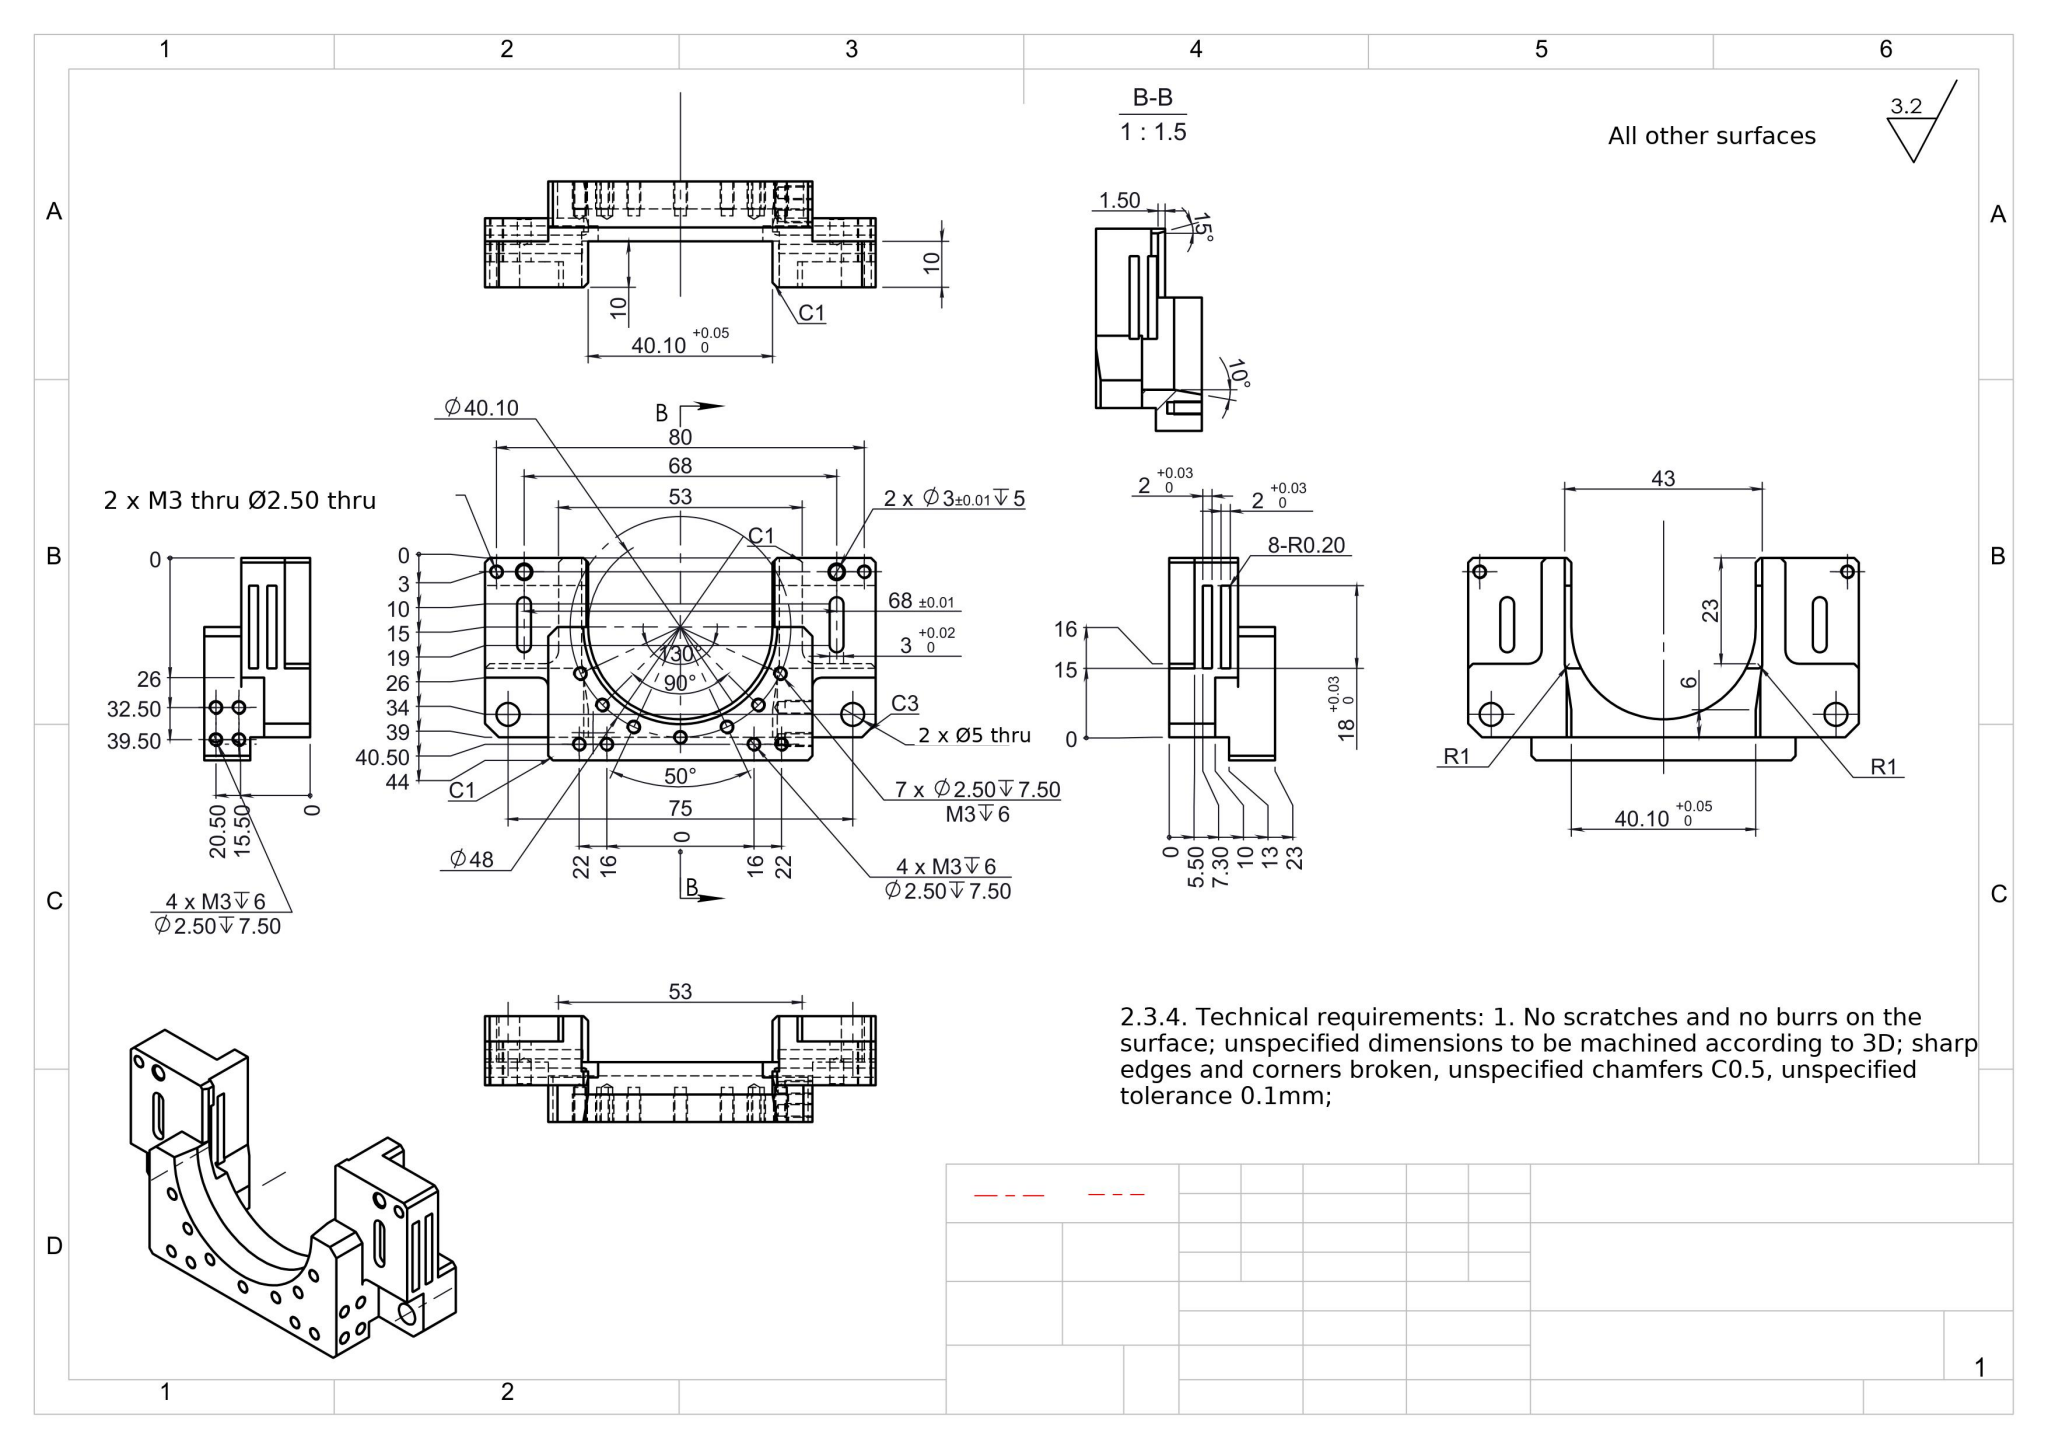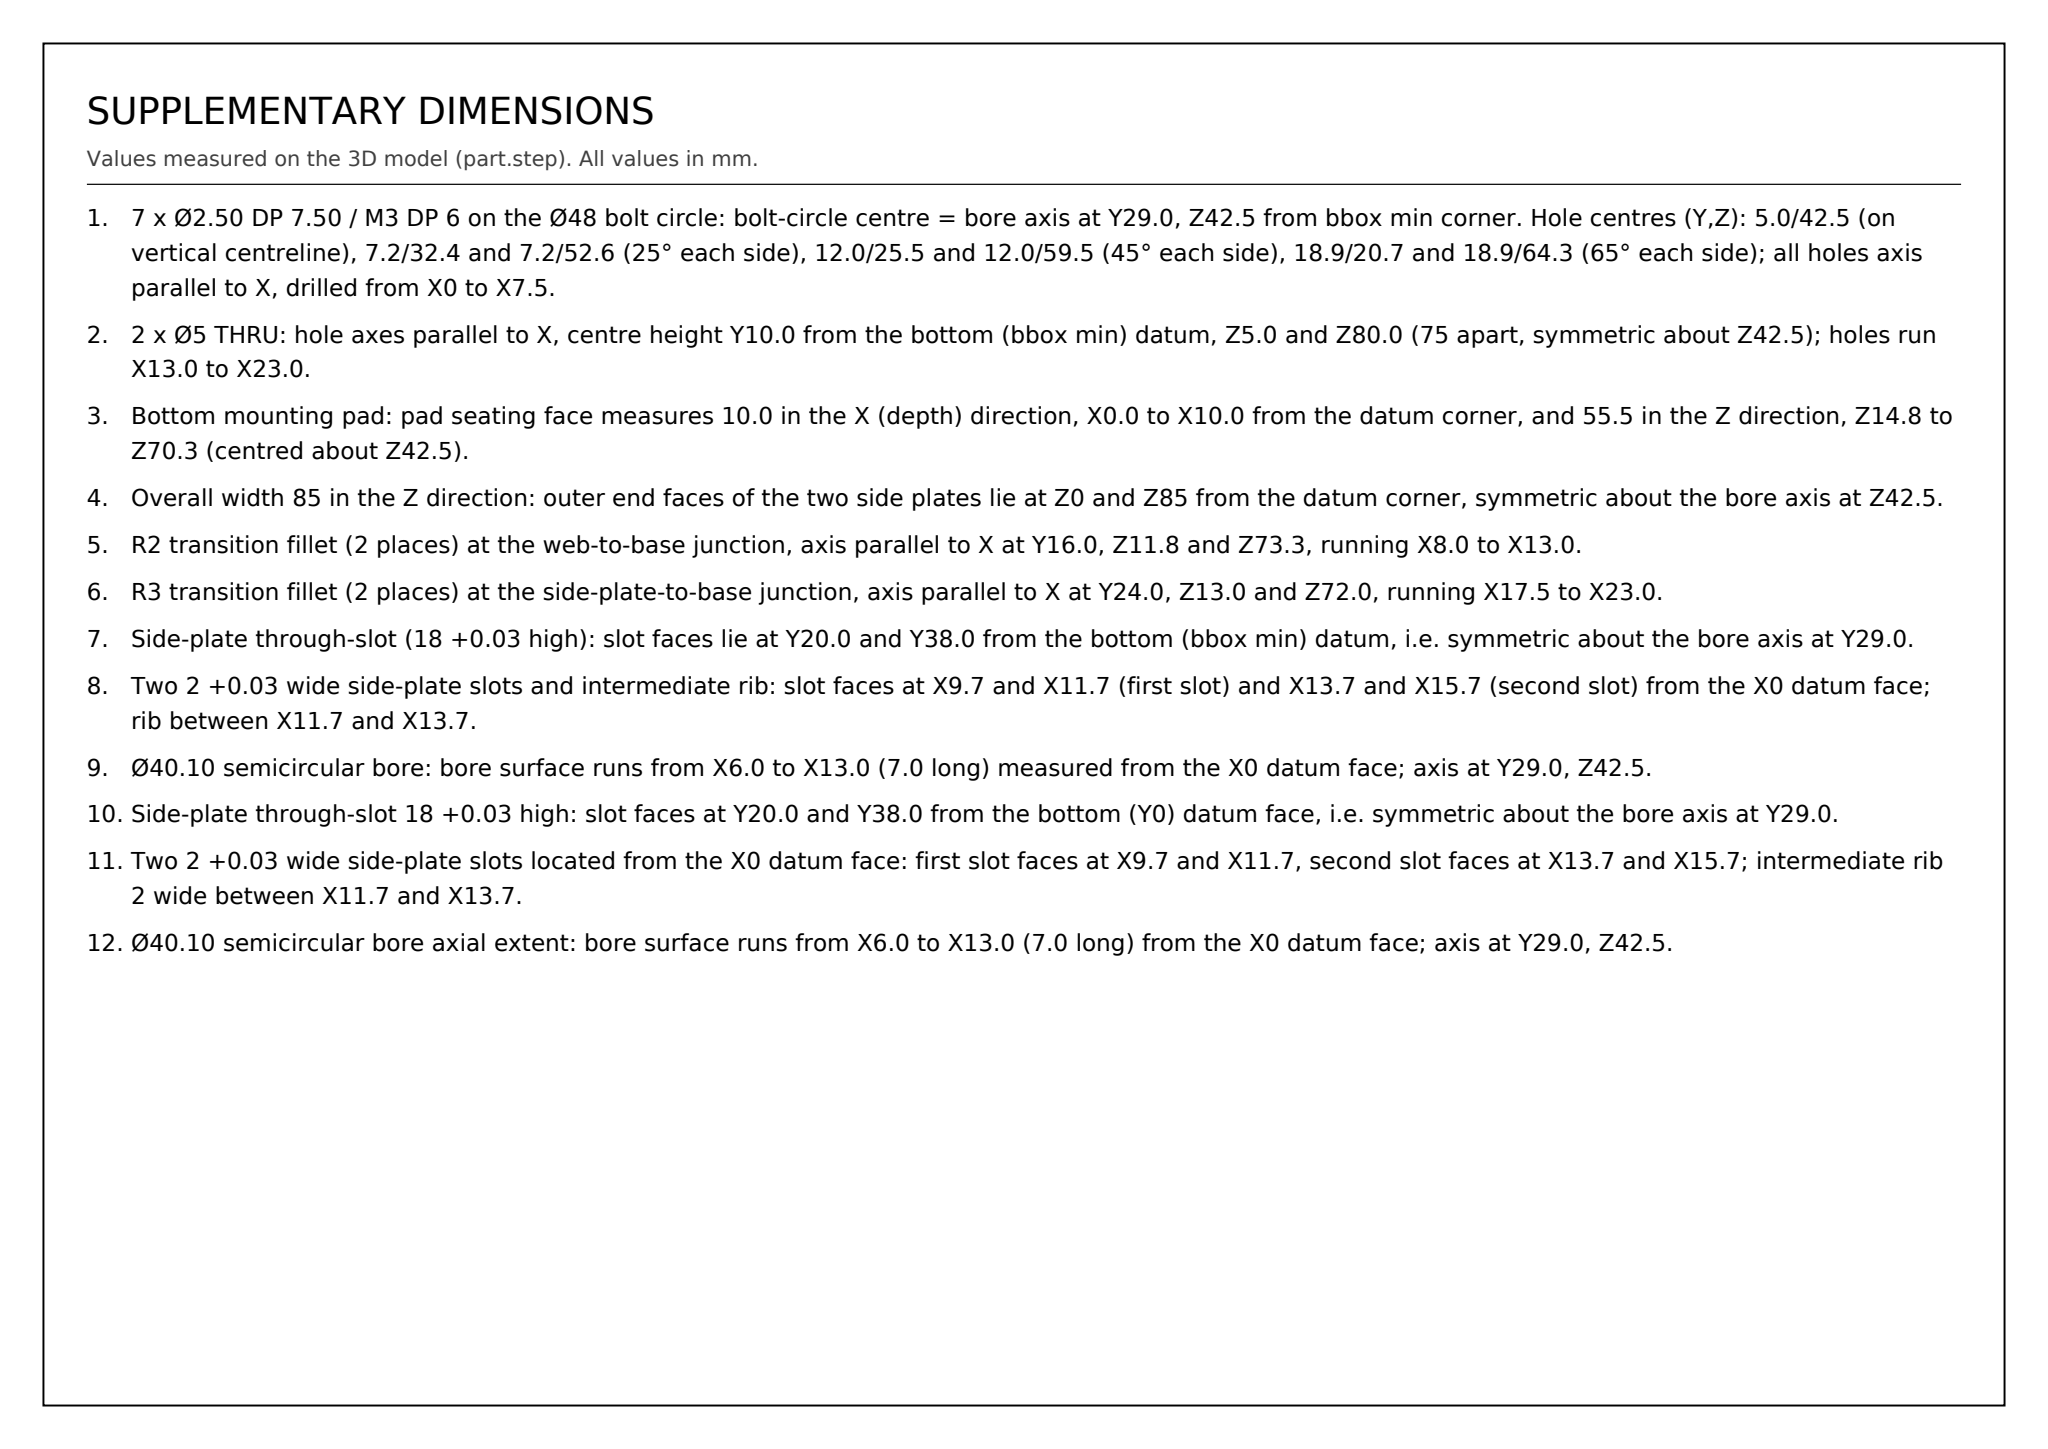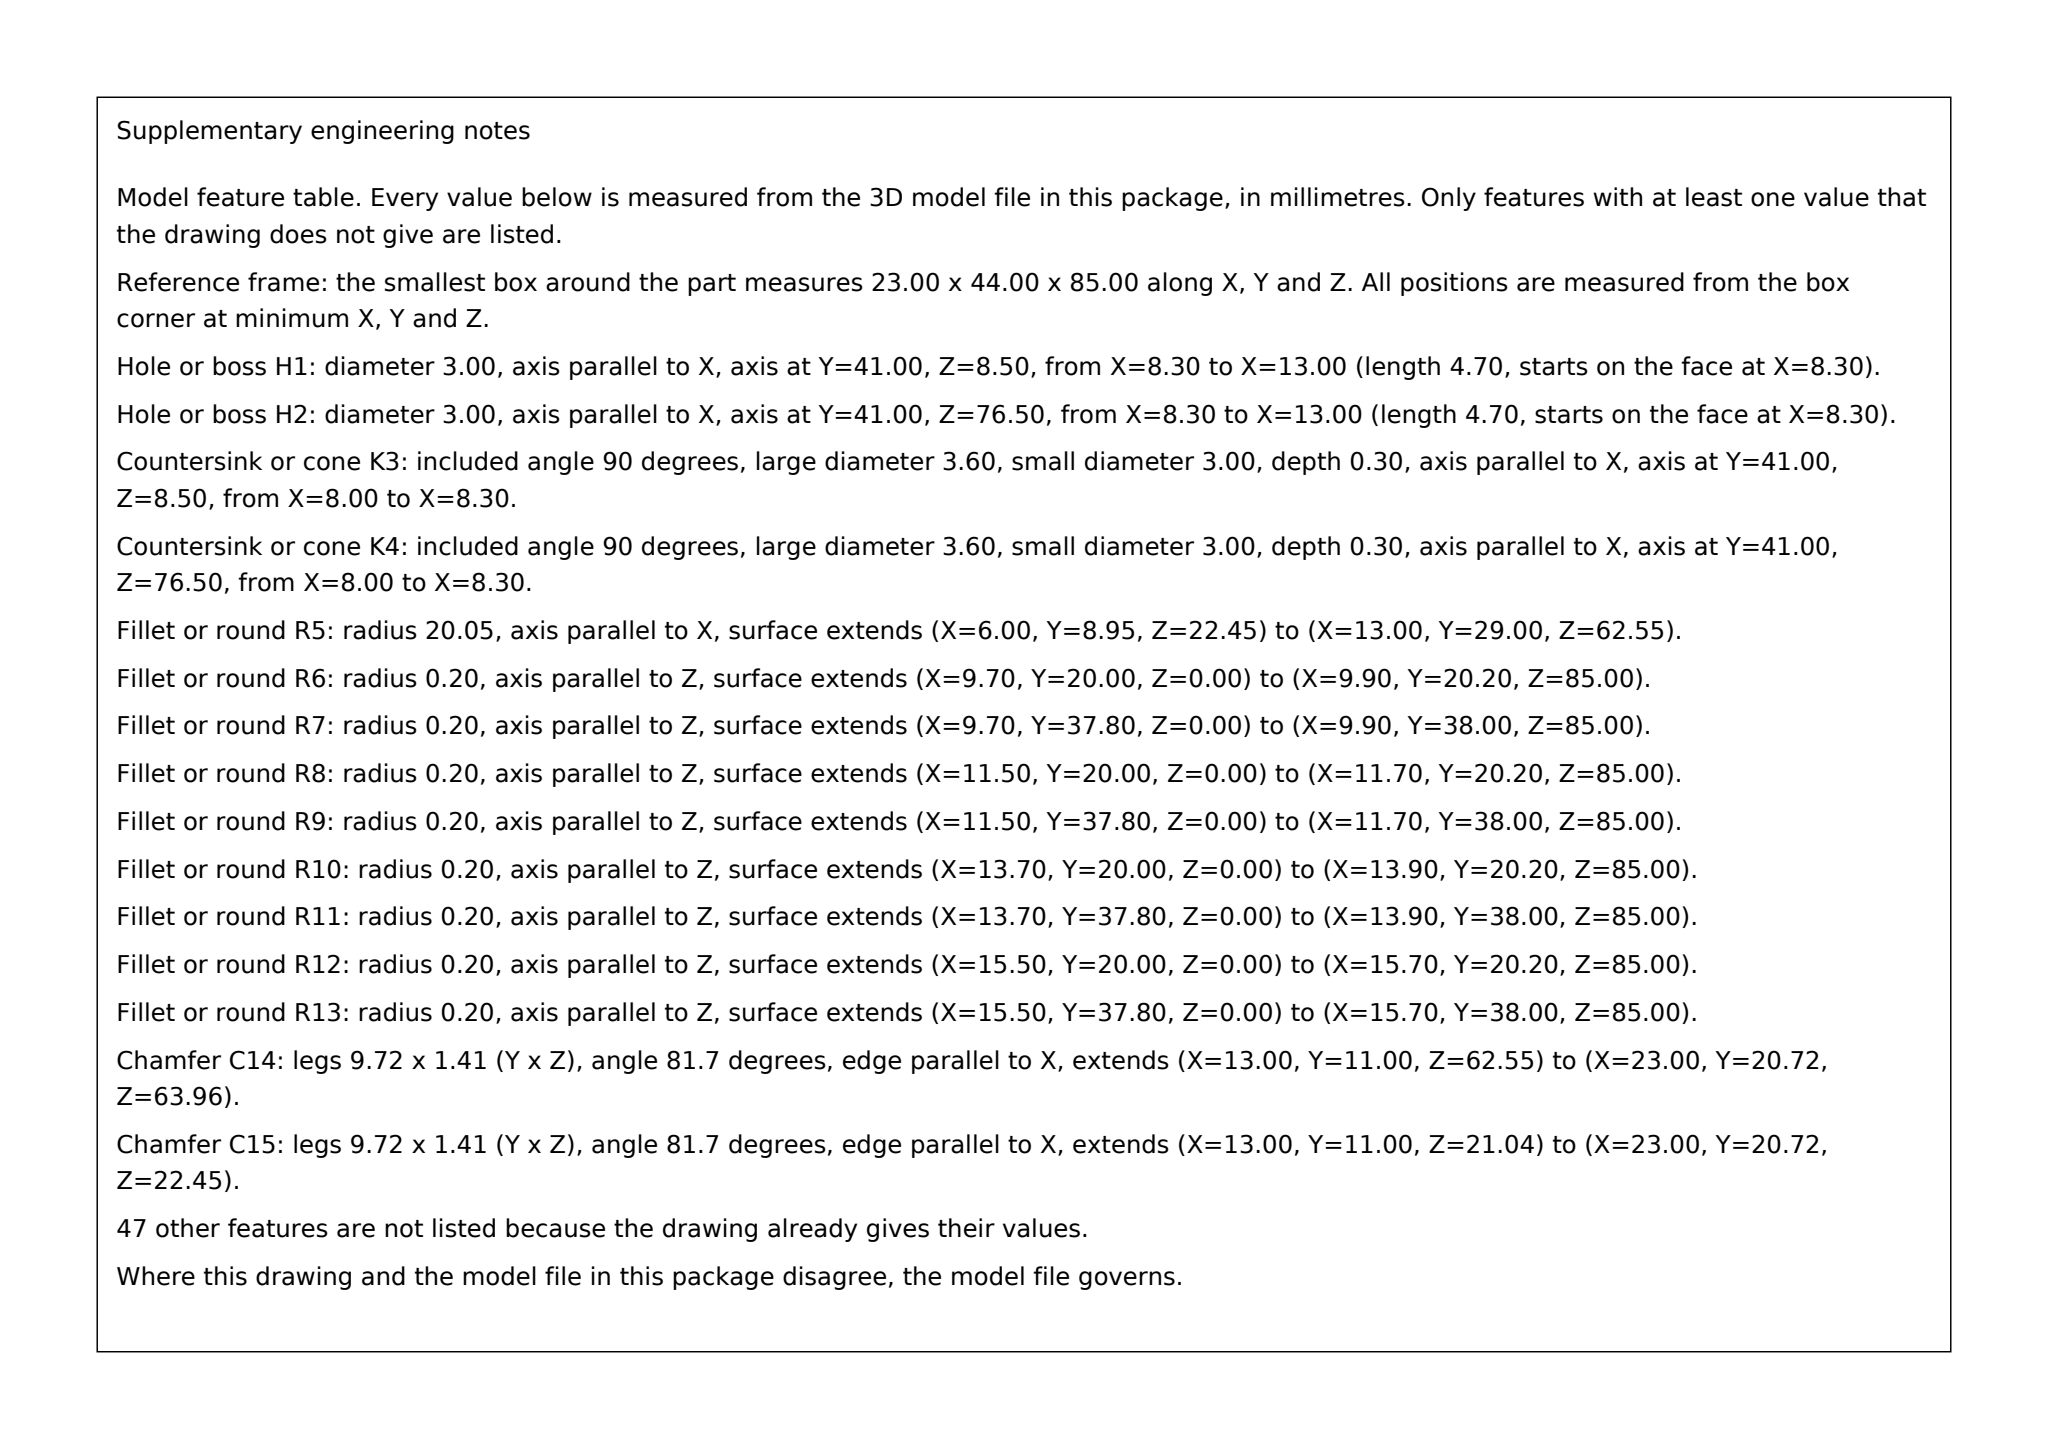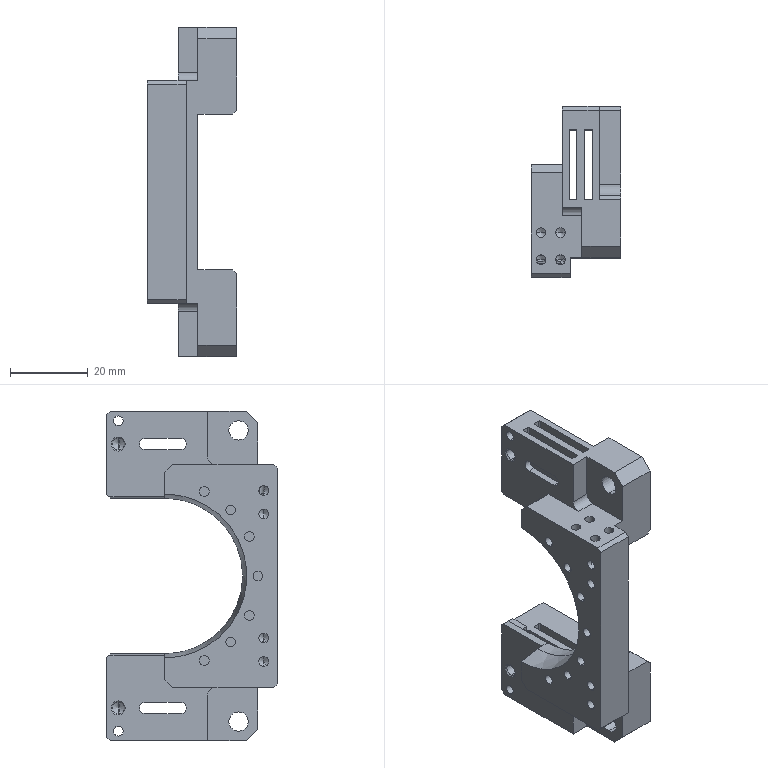Part | SolidWorks | mm | 1 solid | 195 faces | box 23 x 44 x 85 mm | volume 25032 mm3 | plane 90 | cylinder 79 | cone 26 | commonest cylinder face diameters 2.5 x34 3 x16 0.4 x16 5 x4 2 x4 6 x2 4 x2 40.1 x1
Drawing notes:
7 x Ø2.50 DP 7.50 / M3 DP 6 on the Ø48 bolt circle: bolt-circle centre = bore axis at Y29.0, Z42.5 from bbox min corner. Hole centres (Y,Z): 5.0/42.5 (on vertical centreline), 7.2/32.4 and 7.2/52.6 (25° each side), 12.0/25.5 and 12.0/59.5 (45° each side), 18.9/20.7 and 18.9/64.3 (65° each side); all holes axis parallel to X, drilled from X0 to X7.5. | from the solid: hole/bore 2.5 axis x at [y,z] = (5.0,42.5), (7.2,32.4), (7.2,52.6), (12.0,25.5), (12.0,59.5), (18.9,20.7), (18.9,64.3), from 0.0 to 7.5; bore 40.1 axis x at y29.0,z42.5 (bolt-circle/bore centre)
2 x Ø5 THRU: hole axes parallel to X, centre height Y10.0 from the bottom (bbox min) datum, Z5.0 and Z80.0 (75 apart, symmetric about Z42.5); holes run X13.0 to X23.0. | from the solid: hole/bore 5.0 axis x at [null,10.0,5.0] and [null,10.0,80.0], from 13.0 to 23.0
Bottom mounting pad: pad seating face measures 10.0 in the X (depth) direction, X0.0 to X10.0 from the datum corner, and 55.5 in the Z direction, Z14.8 to Z70.3 (centred about Z42.5). | from the solid: planar face normal y at offset 0.0, extent x [0.0, 10.0], z [14.8, 70.3], area 555
Overall width 85 in the Z direction: outer end faces of the two side plates lie at Z0 and Z85 from the datum corner, symmetric about the bore axis at Z42.5. | from the solid: bbox_xyz [23.0, 44.0, 85.0]; axis_planes x=23.0 extents z [0.0,21.5] and z [63.6,85.0]
R2 transition fillet (2 places) at the web-to-base junction, axis parallel to X at Y16.0, Z11.8 and Z73.3, running X8.0 to X13.0. | from the solid: cylinders: concave arc dia 4.0, axis x, [null,16.0,11.8] and [null,16.0,73.3], from 8.0 to 13.0, arc 90
R3 transition fillet (2 places) at the side-plate-to-base junction, axis parallel to X at Y24.0, Z13.0 and Z72.0, running X17.5 to X23.0. | from the solid: cylinders: concave arc dia 6.0, axis x, [null,24.0,13.0] and [null,24.0,72.0], from 17.5 to 23.0, arc 90
Side-plate through-slot (18 +0.03 high): slot faces lie at Y20.0 and Y38.0 from the bottom (bbox min) datum, i.e. symmetric about the bore axis at Y29.0. | from the solid: axis_planes normal y at offset 20.0 and 38.0, extent x[13.9,15.5], z[0,21.1]/[63.9,85.0]; bore cylinder dia 40.1 axis x at y29.0
Two 2 +0.03 wide side-plate slots and intermediate rib: slot faces at X9.7 and X11.7 (first slot) and X13.7 and X15.7 (second slot) from the X0 datum face; rib between X11.7 and X13.7. | from the solid: axis_planes normal x at offsets 9.7, 11.7, 13.7, 15.7, each extent y[20.2,37.8], z[0,21.1]/[63.9,85.0]
Ø40.10 semicircular bore: bore surface runs from X6.0 to X13.0 (7.0 long) measured from the X0 datum face; axis at Y29.0, Z42.5. | from the solid: cylinder dia 40.1, axis x at [y29.0, z42.5], from 6.0 to 13.0, arc 180 deg
Side-plate through-slot 18 +0.03 high: slot faces at Y20.0 and Y38.0 from the bottom (Y0) datum face, i.e. symmetric about the bore axis at Y29.0. | from the solid: axis_planes normal y at offset 20.0 and 38.0 (x 9.9-15.5, z 0-24.6 / 60.4-85.0) - slot top/bottom faces, bore cylinder Ø40.1 axis at y29.0
Two 2 +0.03 wide side-plate slots located from the X0 datum face: first slot faces at X9.7 and X11.7, second slot faces at X13.7 and X15.7; intermediate rib 2 wide between X11.7 and X13.7. | from the solid: axis_planes normal x at offsets 9.7, 11.7, 13.7, 15.7 (y 20.2-37.8) - slot side faces and rib faces
Ø40.10 semicircular bore axial extent: bore surface runs from X6.0 to X13.0 (7.0 long) from the X0 datum face; axis at Y29.0, Z42.5. | from the solid: cylinder 'concave arc' dia 40.1, axis x at (y29.0, z42.5), from 6.0 to 13.0, 180 deg